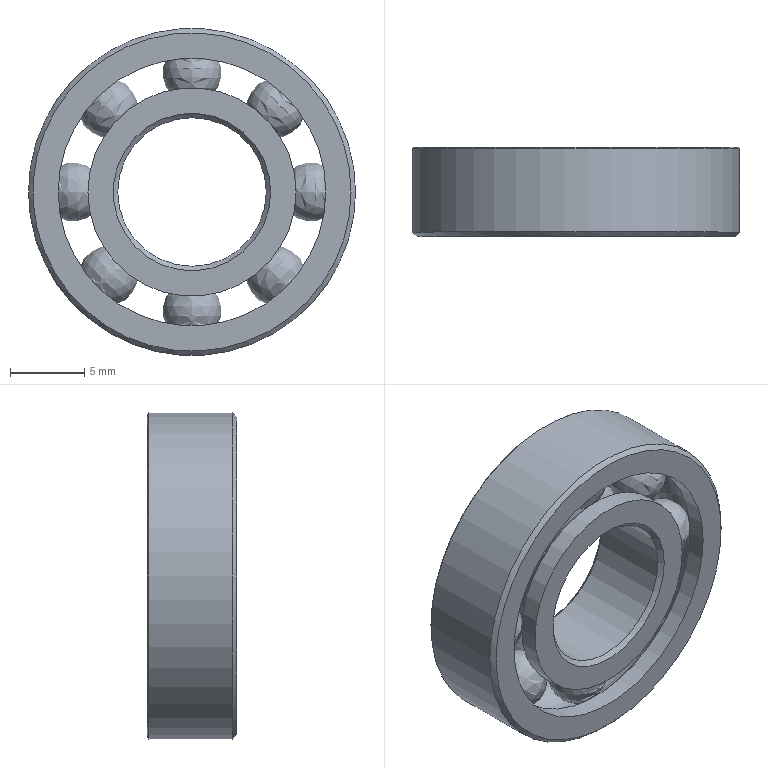Component | NX | GB-T292_AC-1994_71900_AC | 10 solids | 24 faces | volume 1207 mm3 | sphere 8 | cylinder 5 | cone 5 | plane 4 | torus 2 | commonest cylinder face diameters 14 x2 22 x1 18 x1 10 x1